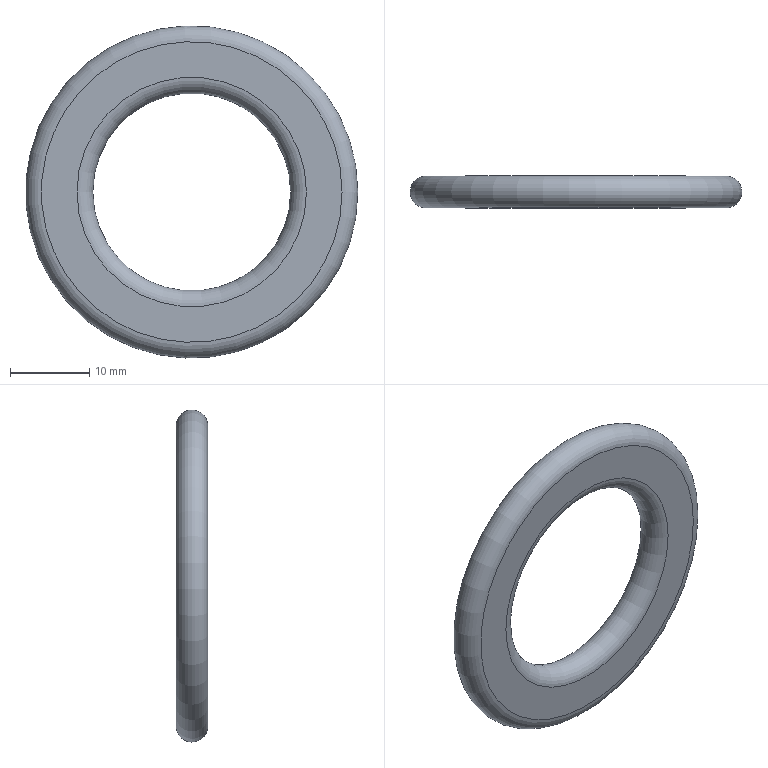Component | NX | 7 | 1 solid | 4 faces | box 42 x 4 x 42 mm | volume 3217 mm3 | plane 2 | torus 2
STEP:
#1=CARTESIAN_POINT('',(0.,0.,0.));
#2=DIRECTION('',(0.,0.,1.));
#3=DIRECTION('',(1.,0.,0.));
#4=AXIS2_PLACEMENT_3D('',#1,#2,#3);
#5=CARTESIAN_POINT('',(-207.317,-37.609,100.));
#6=VERTEX_POINT('',#5);
#7=CARTESIAN_POINT('',(-221.817,-37.609,100.));
#8=DIRECTION('',(0.,-1.,0.));
#9=DIRECTION('',(1.,0.,0.));
#10=AXIS2_PLACEMENT_3D('',#7,#8,#9);
#11=CIRCLE('',#10,14.5);
#12=CARTESIAN_POINT('',(-221.817,-37.609,100.));
#13=DIRECTION('',(0.,1.,0.));
#14=DIRECTION('',(1.,0.,0.));
#15=AXIS2_PLACEMENT_3D('',#12,#13,#14);
#16=PLANE('',#15);
#17=CARTESIAN_POINT('',(14.5,0.));
#18=CARTESIAN_POINT('',(14.5,-25.115));
#19=CARTESIAN_POINT('',(-7.25,-12.557));
#20=CARTESIAN_POINT('',(-29.,-0.));
#21=CARTESIAN_POINT('',(-7.25,12.557));
#22=CARTESIAN_POINT('',(14.5,25.115));
#23=CARTESIAN_POINT('',(14.5,0.));
#24=(BOUNDED_CURVE()B_SPLINE_CURVE(2,(#17,#18,#19,#20,#21,#22,#23),.UNSPECIFIED.,.T.,.F.)B_SPLINE_CURVE_WITH_KNOTS((1,2,2,2,2,1),(-2.094,0.,2.094,4.189,6.283,8.378),.UNSPECIFIED.)CURVE()GEOMETRIC_REPRESENTATION_ITEM()RATIONAL_B_SPLINE_CURVE((1.,0.5,1.,0.5,1.,0.5,1.))REPRESENTATION_ITEM(''));
#25=(GEOMETRIC_REPRESENTATION_CONTEXT(2)PARAMETRIC_REPRESENTATION_CONTEXT()REPRESENTATION_CONTEXT('',''));
#26=DEFINITIONAL_REPRESENTATION('',(#24),#25);
#27=PCURVE('',#16,#26);
#28=CARTESIAN_POINT('',(-221.817,-39.609,100.));
#29=DIRECTION('',(0.,1.,0.));
#30=DIRECTION('',(1.,0.,0.));
#31=AXIS2_PLACEMENT_3D('',#28,#29,#30);
#32=TOROIDAL_SURFACE('',#31,14.5,2.);
#33=CARTESIAN_POINT('',(6.283,1.571));
#34=DIRECTION('',(-1.,0.));
#35=VECTOR('',#34,1.);
#36=LINE('',#33,#35);
#37=(GEOMETRIC_REPRESENTATION_CONTEXT(2)PARAMETRIC_REPRESENTATION_CONTEXT()REPRESENTATION_CONTEXT('',''));
#38=DEFINITIONAL_REPRESENTATION('',(#36),#37);
#39=PCURVE('',#32,#38);
#40=SURFACE_CURVE('',#11,(#27,#39),.PCURVE_S1.);
#41=EDGE_CURVE('',#6,#6,#40,.T.);
#42=ORIENTED_EDGE('',*,*,#41,.T.);
#43=EDGE_LOOP('',(#42));
#44=FACE_BOUND('',#43,.T.);
#45=CARTESIAN_POINT('',(-202.817,-37.609,100.));
#46=VERTEX_POINT('',#45);
#47=CARTESIAN_POINT('',(-221.817,-37.609,100.));
#48=DIRECTION('',(0.,1.,0.));
#49=DIRECTION('',(1.,0.,0.));
#50=AXIS2_PLACEMENT_3D('',#47,#48,#49);
#51=CIRCLE('',#50,19.);
#52=CARTESIAN_POINT('',(0.,0.));
#53=DIRECTION('',(1.,0.));
#54=AXIS2_PLACEMENT_2D('',#52,#53);
#55=CIRCLE('',#54,19.);
#56=(GEOMETRIC_REPRESENTATION_CONTEXT(2)PARAMETRIC_REPRESENTATION_CONTEXT()REPRESENTATION_CONTEXT('',''));
#57=DEFINITIONAL_REPRESENTATION('',(#55),#56);
#58=PCURVE('',#16,#57);
#59=CARTESIAN_POINT('',(-221.817,-39.609,100.));
#60=DIRECTION('',(0.,1.,0.));
#61=DIRECTION('',(1.,0.,0.));
#62=AXIS2_PLACEMENT_3D('',#59,#60,#61);
#63=TOROIDAL_SURFACE('',#62,19.,2.);
#64=CARTESIAN_POINT('',(0.,7.854));
#65=DIRECTION('',(1.,0.));
#66=VECTOR('',#65,1.);
#67=LINE('',#64,#66);
#68=(GEOMETRIC_REPRESENTATION_CONTEXT(2)PARAMETRIC_REPRESENTATION_CONTEXT()REPRESENTATION_CONTEXT('',''));
#69=DEFINITIONAL_REPRESENTATION('',(#67),#68);
#70=PCURVE('',#63,#69);
#71=SURFACE_CURVE('',#51,(#58,#70),.PCURVE_S1.);
#72=EDGE_CURVE('',#46,#46,#71,.T.);
#73=ORIENTED_EDGE('',*,*,#72,.T.);
#74=EDGE_LOOP('',(#73));
#75=FACE_BOUND('',#74,.T.);
#76=ADVANCED_FACE('',(#44,#75),#16,.T.);
#77=CARTESIAN_POINT('',(-207.317,-41.609,100.));
#78=VERTEX_POINT('',#77);
#79=CARTESIAN_POINT('',(-221.817,-41.609,100.));
#80=DIRECTION('',(0.,1.,0.));
#81=DIRECTION('',(1.,0.,0.));
#82=AXIS2_PLACEMENT_3D('',#79,#80,#81);
#83=CIRCLE('',#82,14.5);
#84=CARTESIAN_POINT('',(-221.817,-41.609,100.));
#85=DIRECTION('',(0.,1.,0.));
#86=DIRECTION('',(1.,0.,0.));
#87=AXIS2_PLACEMENT_3D('',#84,#85,#86);
#88=PLANE('',#87);
#89=CARTESIAN_POINT('',(0.,0.));
#90=DIRECTION('',(1.,0.));
#91=AXIS2_PLACEMENT_2D('',#89,#90);
#92=CIRCLE('',#91,14.5);
#93=(GEOMETRIC_REPRESENTATION_CONTEXT(2)PARAMETRIC_REPRESENTATION_CONTEXT()REPRESENTATION_CONTEXT('',''));
#94=DEFINITIONAL_REPRESENTATION('',(#92),#93);
#95=PCURVE('',#88,#94);
#96=CARTESIAN_POINT('',(0.,4.712));
#97=DIRECTION('',(1.,0.));
#98=VECTOR('',#97,1.);
#99=LINE('',#96,#98);
#100=(GEOMETRIC_REPRESENTATION_CONTEXT(2)PARAMETRIC_REPRESENTATION_CONTEXT()REPRESENTATION_CONTEXT('',''));
#101=DEFINITIONAL_REPRESENTATION('',(#99),#100);
#102=PCURVE('',#32,#101);
#103=SURFACE_CURVE('',#83,(#95,#102),.PCURVE_S1.);
#104=EDGE_CURVE('',#78,#78,#103,.T.);
#105=ORIENTED_EDGE('',*,*,#104,.T.);
#106=EDGE_LOOP('',(#105));
#107=FACE_BOUND('',#106,.T.);
#108=CARTESIAN_POINT('',(-202.817,-41.609,100.));
#109=VERTEX_POINT('',#108);
#110=CARTESIAN_POINT('',(-221.817,-41.609,100.));
#111=DIRECTION('',(0.,-1.,0.));
#112=DIRECTION('',(1.,0.,0.));
#113=AXIS2_PLACEMENT_3D('',#110,#111,#112);
#114=CIRCLE('',#113,19.);
#115=CARTESIAN_POINT('',(19.,0.));
#116=CARTESIAN_POINT('',(19.,-32.909));
#117=CARTESIAN_POINT('',(-9.5,-16.454));
#118=CARTESIAN_POINT('',(-38.,-0.));
#119=CARTESIAN_POINT('',(-9.5,16.454));
#120=CARTESIAN_POINT('',(19.,32.909));
#121=CARTESIAN_POINT('',(19.,0.));
#122=(BOUNDED_CURVE()B_SPLINE_CURVE(2,(#115,#116,#117,#118,#119,#120,#121),.UNSPECIFIED.,.T.,.F.)B_SPLINE_CURVE_WITH_KNOTS((1,2,2,2,2,1),(-2.094,0.,2.094,4.189,6.283,8.378),.UNSPECIFIED.)CURVE()GEOMETRIC_REPRESENTATION_ITEM()RATIONAL_B_SPLINE_CURVE((1.,0.5,1.,0.5,1.,0.5,1.))REPRESENTATION_ITEM(''));
#123=(GEOMETRIC_REPRESENTATION_CONTEXT(2)PARAMETRIC_REPRESENTATION_CONTEXT()REPRESENTATION_CONTEXT('',''));
#124=DEFINITIONAL_REPRESENTATION('',(#122),#123);
#125=PCURVE('',#88,#124);
#126=CARTESIAN_POINT('',(6.283,4.712));
#127=DIRECTION('',(-1.,0.));
#128=VECTOR('',#127,1.);
#129=LINE('',#126,#128);
#130=(GEOMETRIC_REPRESENTATION_CONTEXT(2)PARAMETRIC_REPRESENTATION_CONTEXT()REPRESENTATION_CONTEXT('',''));
#131=DEFINITIONAL_REPRESENTATION('',(#129),#130);
#132=PCURVE('',#63,#131);
#133=SURFACE_CURVE('',#114,(#125,#132),.PCURVE_S1.);
#134=EDGE_CURVE('',#109,#109,#133,.T.);
#135=ORIENTED_EDGE('',*,*,#134,.T.);
#136=EDGE_LOOP('',(#135));
#137=FACE_BOUND('',#136,.T.);
#138=ADVANCED_FACE('',(#107,#137),#88,.F.);
#139=ORIENTED_EDGE('',*,*,#104,.F.);
#140=CARTESIAN_POINT('',(-207.317,-37.609,100.));
#141=CARTESIAN_POINT('',(-208.102,-37.609,100.));
#142=CARTESIAN_POINT('',(-208.887,-37.961,100.));
#143=CARTESIAN_POINT('',(-209.488,-38.666,100.));
#144=CARTESIAN_POINT('',(-209.72,-39.609,100.));
#145=CARTESIAN_POINT('',(-209.488,-40.552,100.));
#146=CARTESIAN_POINT('',(-208.887,-41.256,100.));
#147=CARTESIAN_POINT('',(-208.102,-41.609,100.));
#148=CARTESIAN_POINT('',(-207.317,-41.609,100.));
#149=B_SPLINE_CURVE_WITH_KNOTS('',8,(#140,#141,#142,#143,#144,#145,#146,#147,#148),.UNSPECIFIED.,.F.,.F.,(9,9),(1.571,4.712),.PIECEWISE_BEZIER_KNOTS.);
#150=CARTESIAN_POINT('',(0.,0.));
#151=DIRECTION('',(0.,1.));
#152=VECTOR('',#151,1.);
#153=LINE('',#150,#152);
#154=(GEOMETRIC_REPRESENTATION_CONTEXT(2)PARAMETRIC_REPRESENTATION_CONTEXT()REPRESENTATION_CONTEXT('',''));
#155=DEFINITIONAL_REPRESENTATION('',(#153),#154);
#156=PCURVE('',#32,#155);
#157=CARTESIAN_POINT('',(6.283,0.));
#158=DIRECTION('',(0.,1.));
#159=VECTOR('',#158,1.);
#160=LINE('',#157,#159);
#161=(GEOMETRIC_REPRESENTATION_CONTEXT(2)PARAMETRIC_REPRESENTATION_CONTEXT()REPRESENTATION_CONTEXT('',''));
#162=DEFINITIONAL_REPRESENTATION('',(#160),#161);
#163=PCURVE('',#32,#162);
#164=SEAM_CURVE('',#149,(#156,#163),.PCURVE_S1.);
#165=EDGE_CURVE('',#6,#78,#164,.T.);
#166=ORIENTED_EDGE('',*,*,#165,.F.);
#167=ORIENTED_EDGE('',*,*,#41,.F.);
#168=ORIENTED_EDGE('',*,*,#165,.T.);
#169=EDGE_LOOP('',(#139,#166,#167,#168));
#170=FACE_BOUND('',#169,.T.);
#171=ADVANCED_FACE('',(#170),#32,.T.);
#172=ORIENTED_EDGE('',*,*,#72,.F.);
#173=CARTESIAN_POINT('',(-202.817,-41.609,100.));
#174=CARTESIAN_POINT('',(-202.031,-41.609,100.));
#175=CARTESIAN_POINT('',(-201.246,-41.256,100.));
#176=CARTESIAN_POINT('',(-200.645,-40.552,100.));
#177=CARTESIAN_POINT('',(-200.413,-39.609,100.));
#178=CARTESIAN_POINT('',(-200.645,-38.666,100.));
#179=CARTESIAN_POINT('',(-201.246,-37.961,100.));
#180=CARTESIAN_POINT('',(-202.031,-37.609,100.));
#181=CARTESIAN_POINT('',(-202.817,-37.609,100.));
#182=B_SPLINE_CURVE_WITH_KNOTS('',8,(#173,#174,#175,#176,#177,#178,#179,#180,#181),.UNSPECIFIED.,.F.,.F.,(9,9),(-1.571,1.571),.PIECEWISE_BEZIER_KNOTS.);
#183=CARTESIAN_POINT('',(0.,6.283));
#184=DIRECTION('',(0.,1.));
#185=VECTOR('',#184,1.);
#186=LINE('',#183,#185);
#187=(GEOMETRIC_REPRESENTATION_CONTEXT(2)PARAMETRIC_REPRESENTATION_CONTEXT()REPRESENTATION_CONTEXT('',''));
#188=DEFINITIONAL_REPRESENTATION('',(#186),#187);
#189=PCURVE('',#63,#188);
#190=CARTESIAN_POINT('',(6.283,6.283));
#191=DIRECTION('',(0.,1.));
#192=VECTOR('',#191,1.);
#193=LINE('',#190,#192);
#194=(GEOMETRIC_REPRESENTATION_CONTEXT(2)PARAMETRIC_REPRESENTATION_CONTEXT()REPRESENTATION_CONTEXT('',''));
#195=DEFINITIONAL_REPRESENTATION('',(#193),#194);
#196=PCURVE('',#63,#195);
#197=SEAM_CURVE('',#182,(#189,#196),.PCURVE_S1.);
#198=EDGE_CURVE('',#109,#46,#197,.T.);
#199=ORIENTED_EDGE('',*,*,#198,.F.);
#200=ORIENTED_EDGE('',*,*,#134,.F.);
#201=ORIENTED_EDGE('',*,*,#198,.T.);
#202=EDGE_LOOP('',(#172,#199,#200,#201));
#203=FACE_BOUND('',#202,.T.);
#204=ADVANCED_FACE('',(#203),#63,.T.);
#205=CLOSED_SHELL('',(#76,#138,#171,#204));
#206=MANIFOLD_SOLID_BREP('',#205);
#207=(LENGTH_UNIT()NAMED_UNIT(*)SI_UNIT(.MILLI.,.METRE.));
#208=UNCERTAINTY_MEASURE_WITH_UNIT(LENGTH_MEASURE(0.00001),#207,'','');
#209=(NAMED_UNIT(*)PLANE_ANGLE_UNIT()SI_UNIT($,.RADIAN.));
#210=(NAMED_UNIT(*)SI_UNIT($,.STERADIAN.)SOLID_ANGLE_UNIT());
#211=(GEOMETRIC_REPRESENTATION_CONTEXT(3)GLOBAL_UNCERTAINTY_ASSIGNED_CONTEXT((#208))GLOBAL_UNIT_ASSIGNED_CONTEXT((#207,#209,#210))REPRESENTATION_CONTEXT('',''));
#212=ADVANCED_BREP_SHAPE_REPRESENTATION('',(#4,#206),#211);